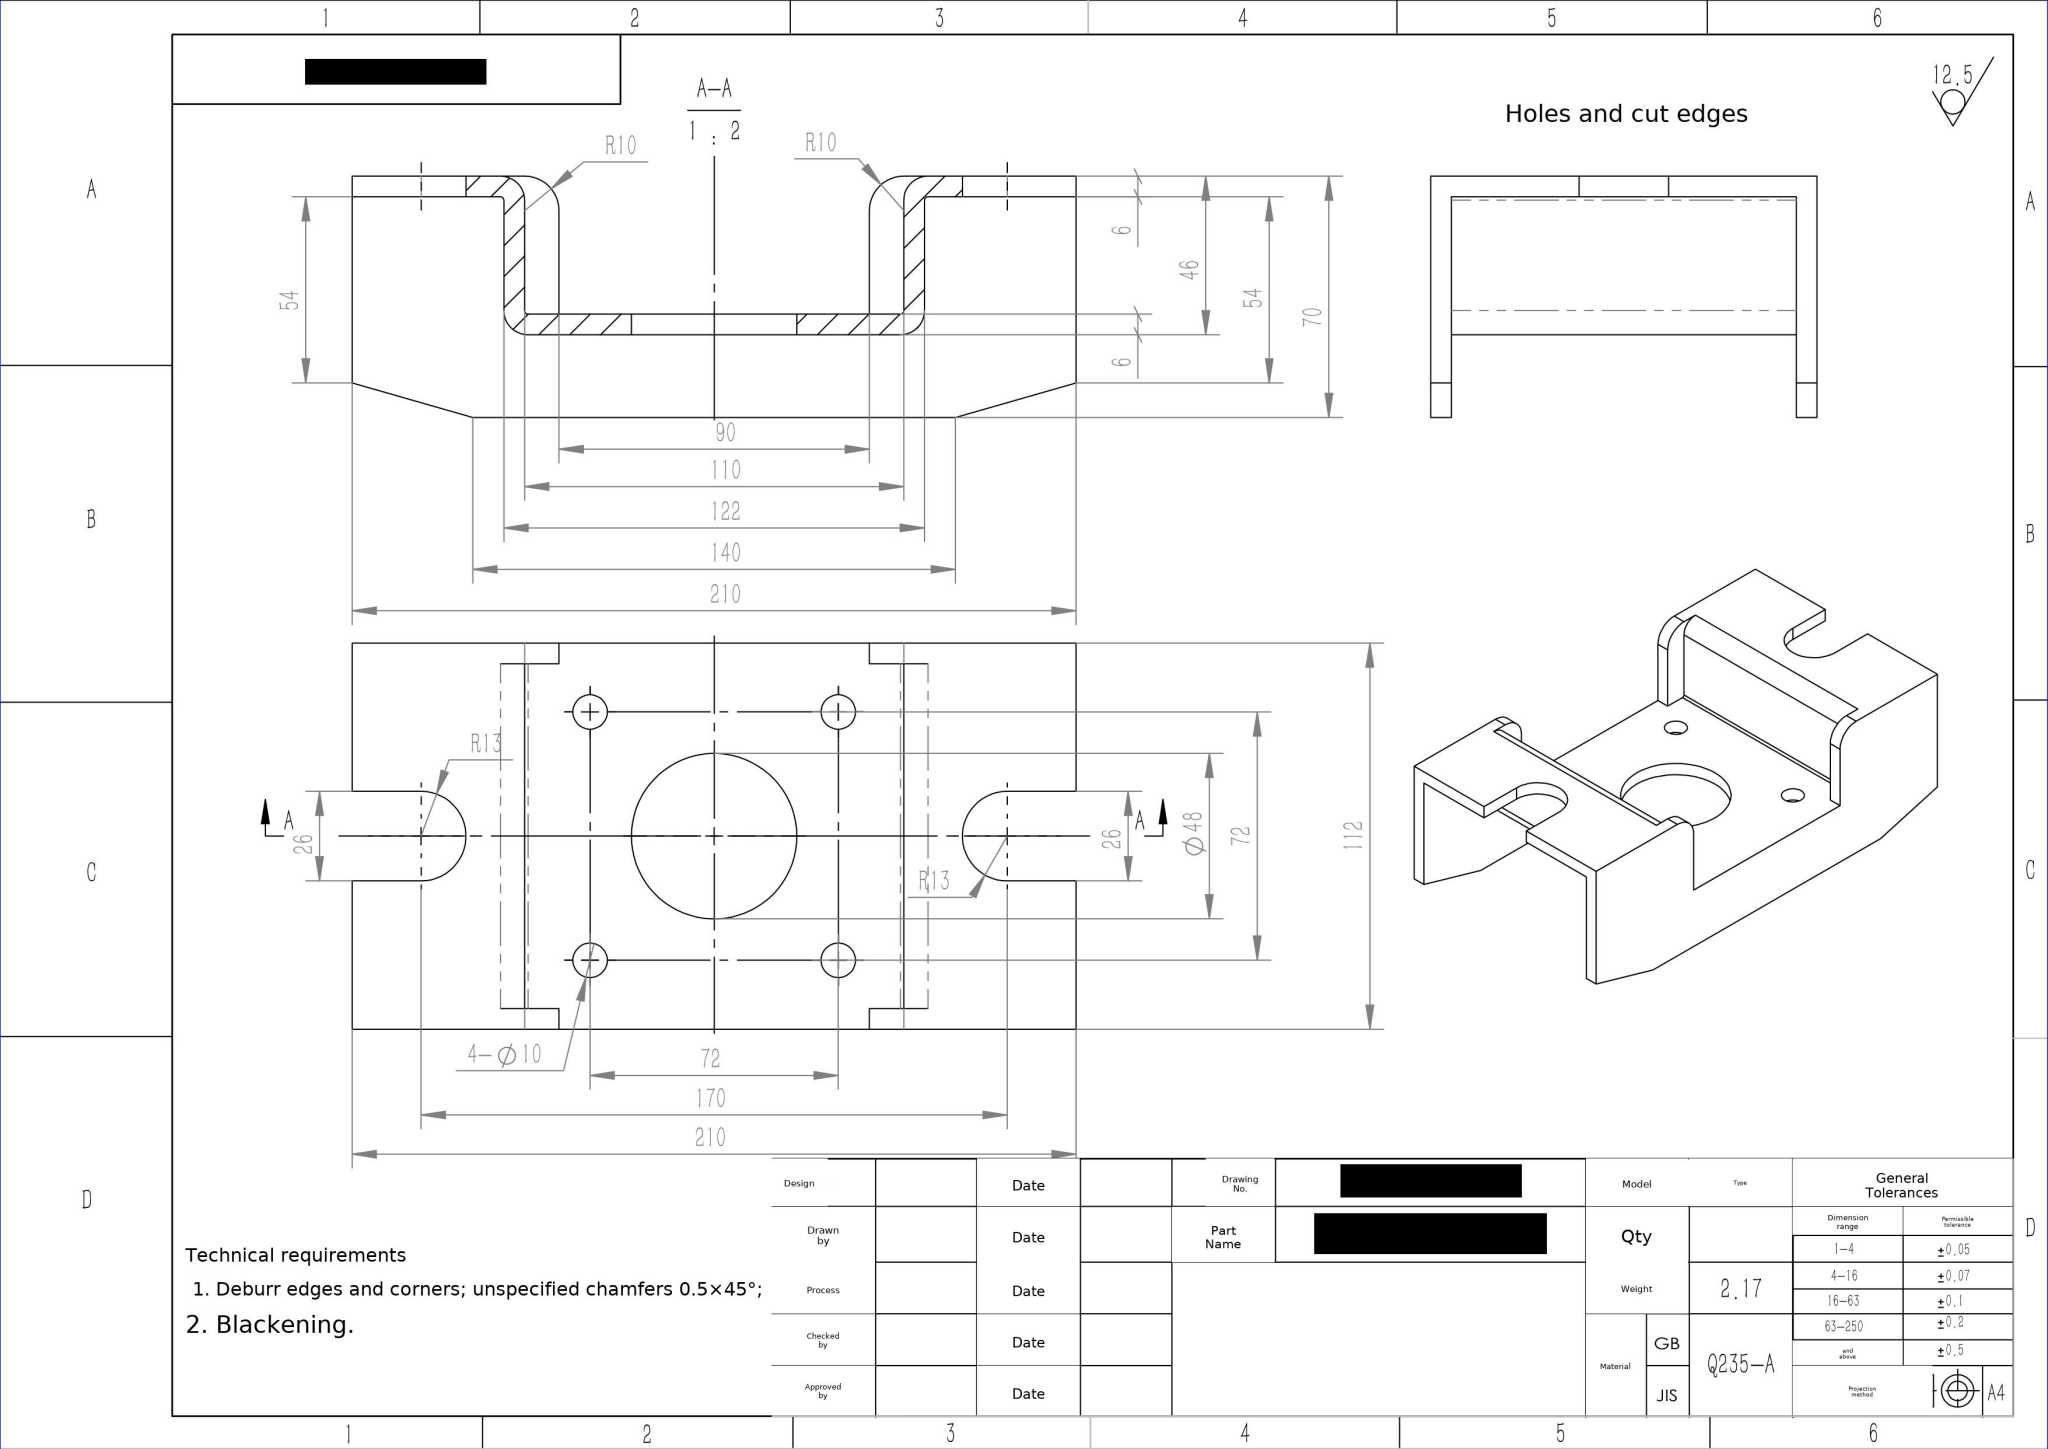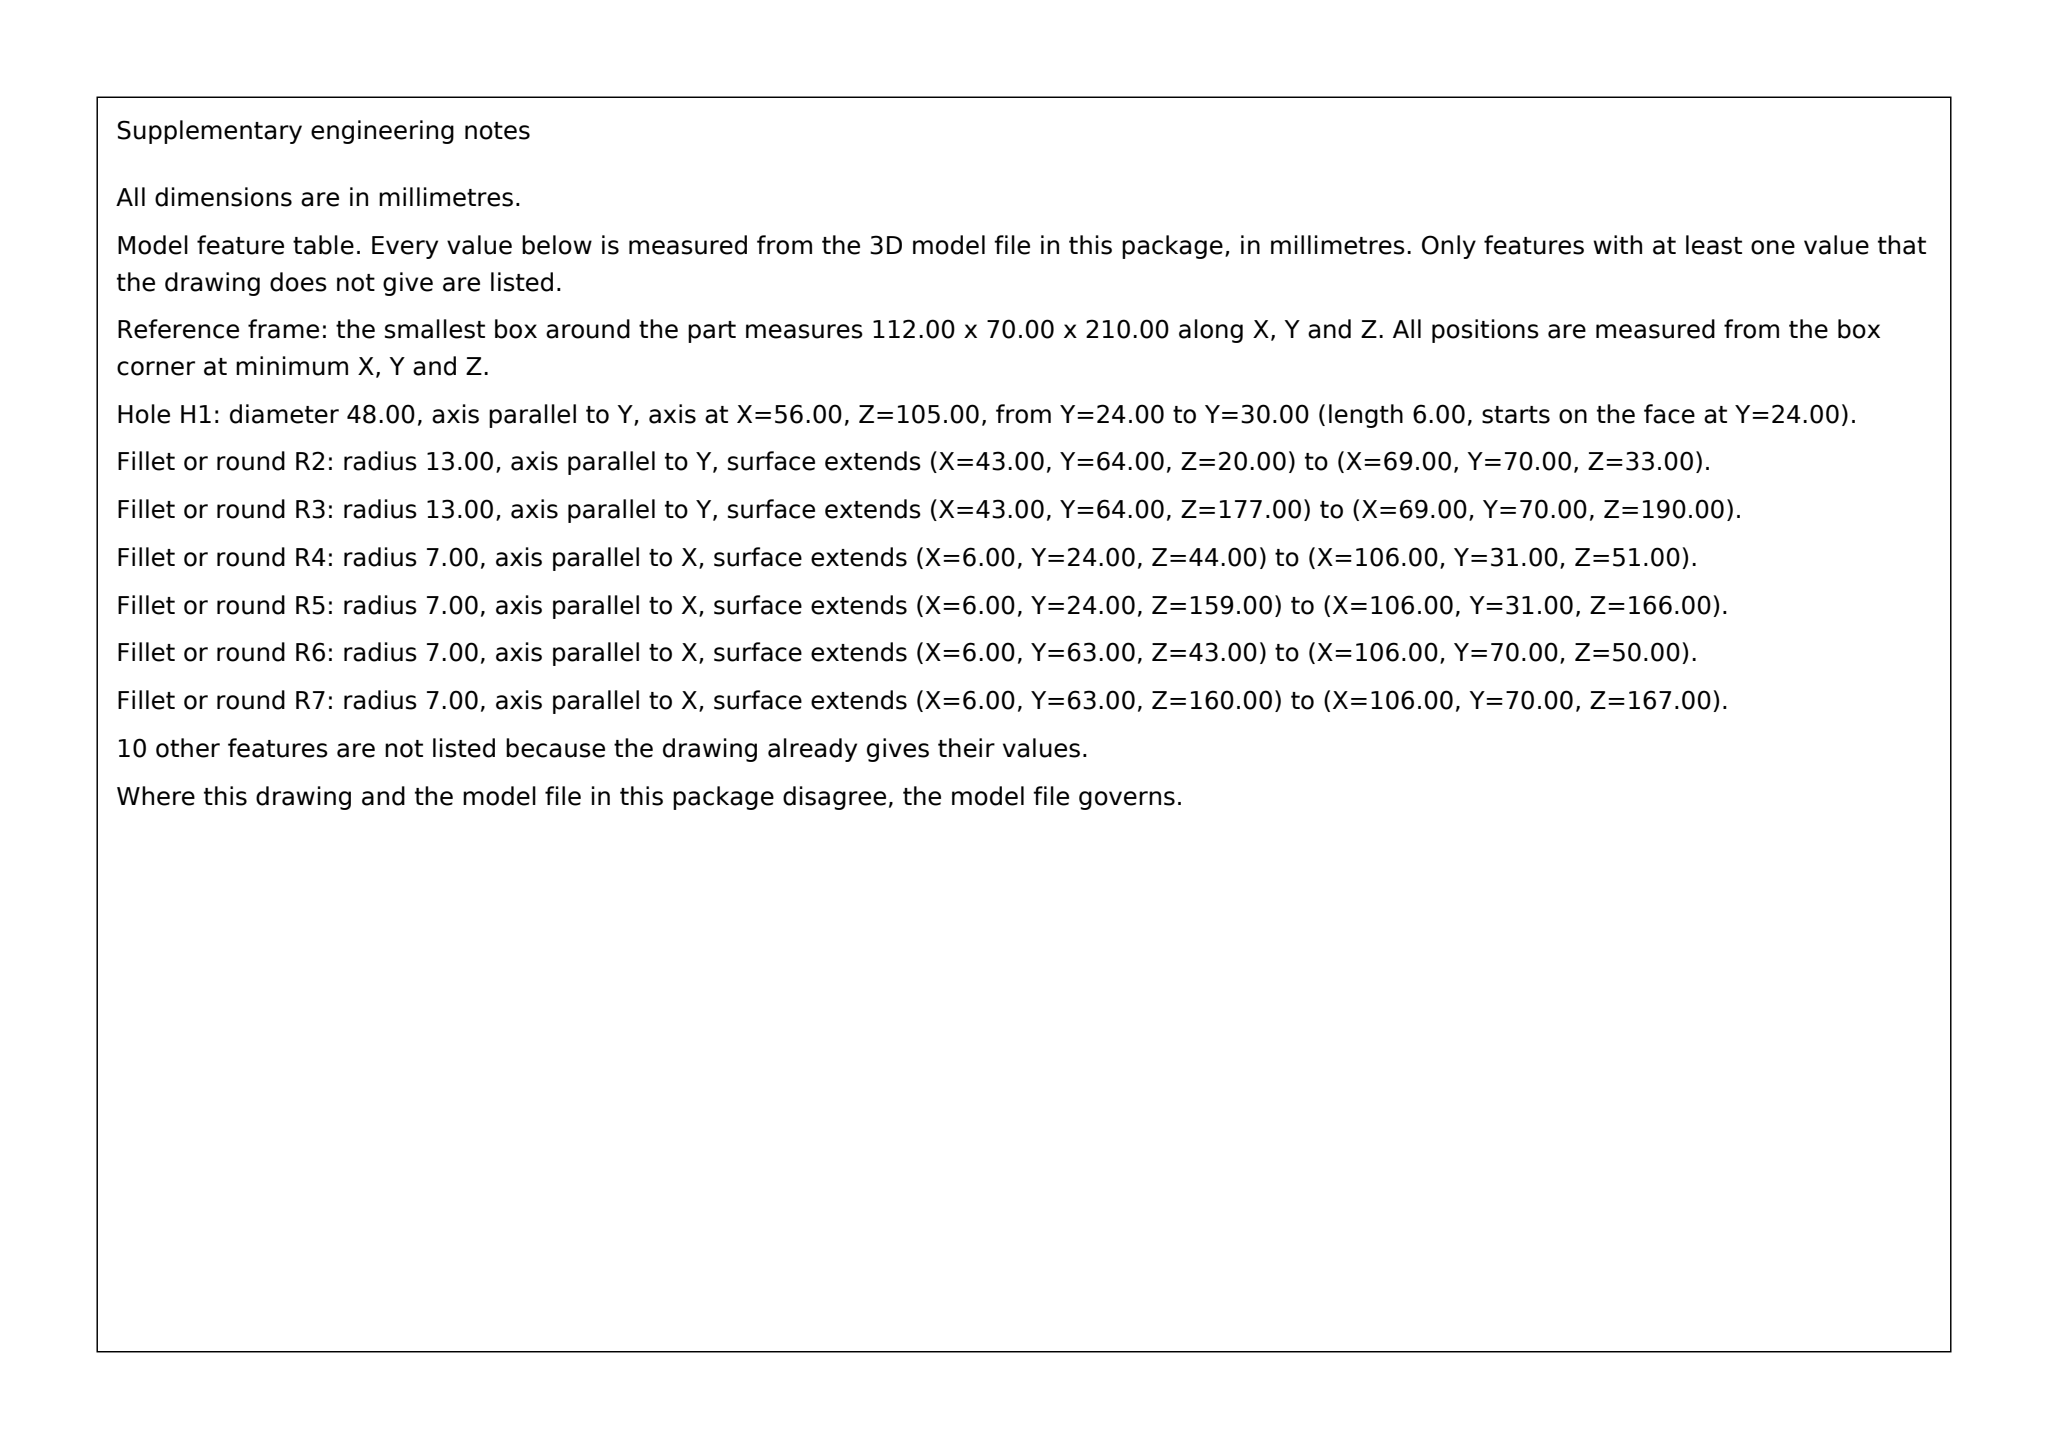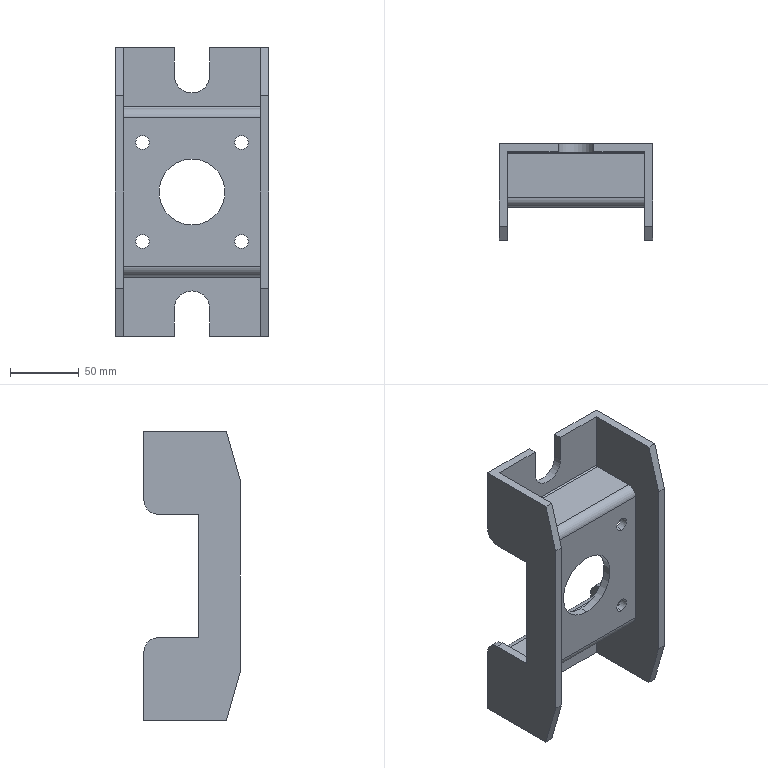Part | SolidWorks | mm | material Q235-A | 1 solid | 61 faces | box 112 x 70 x 210 mm | volume 276197 mm3 | plane 36 | cylinder 25 | commonest cylinder face diameters 10 x8 20 x4 14 x4 2 x4 26 x3 48 x2